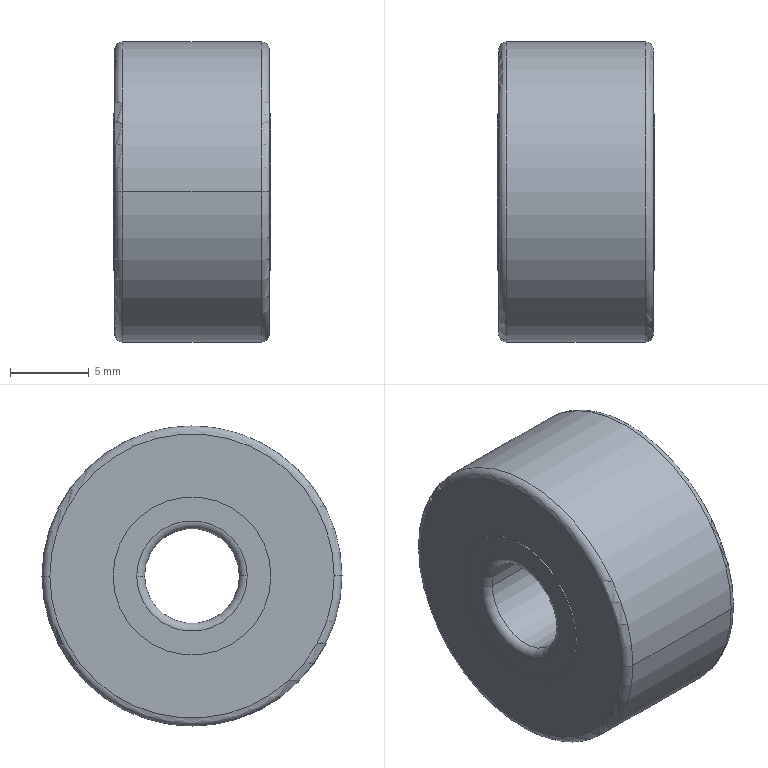Component | SolidWorks | ClampingArm2-1_BPS01-d6-1 | 1 solid | 20 faces | box 10 x 19 x 19 mm | volume 2503 mm3 | torus 8 | cylinder 8 | plane 4 | commonest cylinder face diameters 10 x4 6 x2 19 x2 | material Standard Part
build123d program:
from build123d import *

# Parameters (mm, degrees)
SKETCH1_R           = 9.5
BOSS_EXTRUDE1_DEPTH = 4.9
SKETCH2_R           = 5
BOSS_EXTRUDE2_DEPTH = 5
SKETCH3_R           = 3
CUT_EXTRUDE1_DEPTH  = 17.748
FILLET1_R           = 0.5


with BuildPart() as part:
    # Sketch1 → Boss-Extrude1 (new, symmetric)
    with BuildSketch(Plane(origin=(0, 0, 0), x_dir=(0, 0, -1), z_dir=(1, 0, 0))):
        Circle(SKETCH1_R)
    extrude(amount=BOSS_EXTRUDE1_DEPTH, both=True)

    # Sketch2 → Boss-Extrude2 (add, symmetric)
    with BuildSketch(Plane(origin=(0, 0, 0), x_dir=(0, 0, -1), z_dir=(1, 0, 0))):
        Circle(SKETCH2_R)
    extrude(amount=BOSS_EXTRUDE2_DEPTH, both=True)

    # Sketch3 → Cut-Extrude1 (cut, through all)
    with BuildSketch(Plane(origin=(5, 0, 0), x_dir=(0, 0, -1), z_dir=(1, 0, 0))):
        Circle(SKETCH3_R)
    extrude(amount=-CUT_EXTRUDE1_DEPTH, mode=Mode.SUBTRACT)

    # Fillet1
    fillet1_edges = [part.edges().sort_by_distance(p)[0] for p in [
        (-5, 0, 3),
        (5, 0, 3),
        (-4.9, 0, 9.5),
        (4.9, 0, 9.5),
    ]]
    fillet(fillet1_edges, radius=FILLET1_R)


solid = part.part

# Placed as in the assembly
solid = solid.moved(Location((-7.551, 66.046, -22.5), (0, 0, 0)))
STEP:
#1=COLOUR_RGB('',0.7922,0.8196,0.9333);
#2=FILL_AREA_STYLE_COLOUR('',#1);
#3=FILL_AREA_STYLE('',(#2));
#4=SURFACE_STYLE_FILL_AREA(#3);
#5=SURFACE_SIDE_STYLE('',(#4));
#6=SURFACE_STYLE_USAGE(.BOTH.,#5);
#7=PRESENTATION_STYLE_ASSIGNMENT((#6));
#8=CARTESIAN_POINT('',(-0.124,2.226,-0.8857));
#9=VERTEX_POINT('',#8);
#10=CARTESIAN_POINT('',(-0.124,2.974,-0.886));
#11=VERTEX_POINT('',#10);
#12=CARTESIAN_POINT('',(-0.124,2.6,-0.8858));
#13=DIRECTION('',(-1.,-0.,0.));
#14=DIRECTION('',(-0.,1.,-0.0003333));
#15=AXIS2_PLACEMENT_3D('',#12,#13,#14);
#16=CIRCLE('',#15,0.374);
#17=EDGE_CURVE('',#9,#11,#16,.T.);
#18=ORIENTED_EDGE('',*,*,#17,.F.);
#19=CARTESIAN_POINT('',(-0.1044,2.246,-0.8857));
#20=VERTEX_POINT('',#19);
#21=CARTESIAN_POINT('',(-0.124,2.246,-0.8857));
#22=DIRECTION('',(0.,0.0003333,1.));
#23=DIRECTION('',(0.,-1.,0.0003333));
#24=AXIS2_PLACEMENT_3D('',#21,#22,#23);
#25=CIRCLE('',#24,0.01969);
#26=EDGE_CURVE('',#9,#20,#25,.T.);
#27=ORIENTED_EDGE('',*,*,#26,.T.);
#28=CARTESIAN_POINT('',(-0.1044,2.955,-0.8859));
#29=VERTEX_POINT('',#28);
#30=CARTESIAN_POINT('',(-0.1044,2.6,-0.8858));
#31=DIRECTION('',(1.,0.,-0.));
#32=DIRECTION('',(-0.,1.,-0.0003333));
#33=AXIS2_PLACEMENT_3D('',#30,#31,#32);
#34=CIRCLE('',#33,0.3543);
#35=EDGE_CURVE('',#29,#20,#34,.T.);
#36=ORIENTED_EDGE('',*,*,#35,.F.);
#37=CARTESIAN_POINT('',(-0.124,2.955,-0.8859));
#38=DIRECTION('',(-0.,-0.0003333,-1.));
#39=DIRECTION('',(0.,1.,-0.0003333));
#40=AXIS2_PLACEMENT_3D('',#37,#38,#39);
#41=CIRCLE('',#40,0.01969);
#42=EDGE_CURVE('',#11,#29,#41,.T.);
#43=ORIENTED_EDGE('',*,*,#42,.F.);
#44=EDGE_LOOP('',(#18,#27,#36,#43));
#45=FACE_OUTER_BOUND('',#44,.T.);
#46=CARTESIAN_POINT('',(-0.124,2.6,-0.8858));
#47=DIRECTION('',(1.,0.,-0.));
#48=DIRECTION('',(-0.,1.,-0.0003333));
#49=AXIS2_PLACEMENT_3D('',#46,#47,#48);
#50=TOROIDAL_SURFACE('',#49,0.3543,0.01969);
#51=ADVANCED_FACE('',(#45),#50,.T.);
#52=CARTESIAN_POINT('',(-0.1004,2.462,-0.8858));
#53=VERTEX_POINT('',#52);
#54=CARTESIAN_POINT('',(-0.1004,2.738,-0.8859));
#55=VERTEX_POINT('',#54);
#56=CARTESIAN_POINT('',(-0.1004,2.6,-0.8858));
#57=DIRECTION('',(-1.,-0.,0.));
#58=DIRECTION('',(-0.,1.,-0.0003333));
#59=AXIS2_PLACEMENT_3D('',#56,#57,#58);
#60=CIRCLE('',#59,0.1378);
#61=EDGE_CURVE('',#53,#55,#60,.T.);
#62=ORIENTED_EDGE('',*,*,#61,.F.);
#63=CARTESIAN_POINT('',(-0.1201,2.482,-0.8858));
#64=VERTEX_POINT('',#63);
#65=CARTESIAN_POINT('',(-0.1201,2.462,-0.8858));
#66=DIRECTION('',(0.,0.0003333,1.));
#67=DIRECTION('',(0.,-1.,0.0003333));
#68=AXIS2_PLACEMENT_3D('',#65,#66,#67);
#69=CIRCLE('',#68,0.01969);
#70=EDGE_CURVE('',#53,#64,#69,.T.);
#71=ORIENTED_EDGE('',*,*,#70,.T.);
#72=CARTESIAN_POINT('',(-0.1201,2.718,-0.8859));
#73=VERTEX_POINT('',#72);
#74=CARTESIAN_POINT('',(-0.1201,2.6,-0.8858));
#75=DIRECTION('',(1.,0.,-0.));
#76=DIRECTION('',(-0.,1.,-0.0003333));
#77=AXIS2_PLACEMENT_3D('',#74,#75,#76);
#78=CIRCLE('',#77,0.1181);
#79=EDGE_CURVE('',#73,#64,#78,.T.);
#80=ORIENTED_EDGE('',*,*,#79,.F.);
#81=CARTESIAN_POINT('',(-0.1201,2.738,-0.8859));
#82=DIRECTION('',(-0.,-0.0003333,-1.));
#83=DIRECTION('',(0.,1.,-0.0003333));
#84=AXIS2_PLACEMENT_3D('',#81,#82,#83);
#85=CIRCLE('',#84,0.01969);
#86=EDGE_CURVE('',#55,#73,#85,.T.);
#87=ORIENTED_EDGE('',*,*,#86,.F.);
#88=EDGE_LOOP('',(#62,#71,#80,#87));
#89=FACE_OUTER_BOUND('',#88,.T.);
#90=CARTESIAN_POINT('',(-0.1201,2.6,-0.8858));
#91=DIRECTION('',(1.,0.,-0.));
#92=DIRECTION('',(-0.,1.,-0.0003333));
#93=AXIS2_PLACEMENT_3D('',#90,#91,#92);
#94=TOROIDAL_SURFACE('',#93,0.1378,0.01969);
#95=ADVANCED_FACE('',(#89),#94,.T.);
#96=CARTESIAN_POINT('',(-0.4902,2.246,-0.8857));
#97=VERTEX_POINT('',#96);
#98=CARTESIAN_POINT('',(-0.4902,2.955,-0.8859));
#99=VERTEX_POINT('',#98);
#100=CARTESIAN_POINT('',(-0.4902,2.6,-0.8858));
#101=DIRECTION('',(-1.,-0.,0.));
#102=DIRECTION('',(-0.,1.,-0.0003333));
#103=AXIS2_PLACEMENT_3D('',#100,#101,#102);
#104=CIRCLE('',#103,0.3543);
#105=EDGE_CURVE('',#97,#99,#104,.T.);
#106=ORIENTED_EDGE('',*,*,#105,.F.);
#107=CARTESIAN_POINT('',(-0.4705,2.226,-0.8857));
#108=VERTEX_POINT('',#107);
#109=CARTESIAN_POINT('',(-0.4705,2.246,-0.8857));
#110=DIRECTION('',(0.,0.0003333,1.));
#111=DIRECTION('',(0.,-1.,0.0003333));
#112=AXIS2_PLACEMENT_3D('',#109,#110,#111);
#113=CIRCLE('',#112,0.01969);
#114=EDGE_CURVE('',#97,#108,#113,.T.);
#115=ORIENTED_EDGE('',*,*,#114,.T.);
#116=CARTESIAN_POINT('',(-0.4705,2.974,-0.886));
#117=VERTEX_POINT('',#116);
#118=CARTESIAN_POINT('',(-0.4705,2.6,-0.8858));
#119=DIRECTION('',(1.,0.,-0.));
#120=DIRECTION('',(-0.,1.,-0.0003333));
#121=AXIS2_PLACEMENT_3D('',#118,#119,#120);
#122=CIRCLE('',#121,0.374);
#123=EDGE_CURVE('',#117,#108,#122,.T.);
#124=ORIENTED_EDGE('',*,*,#123,.F.);
#125=CARTESIAN_POINT('',(-0.4705,2.955,-0.8859));
#126=DIRECTION('',(-0.,-0.0003333,-1.));
#127=DIRECTION('',(0.,1.,-0.0003333));
#128=AXIS2_PLACEMENT_3D('',#125,#126,#127);
#129=CIRCLE('',#128,0.01969);
#130=EDGE_CURVE('',#99,#117,#129,.T.);
#131=ORIENTED_EDGE('',*,*,#130,.F.);
#132=EDGE_LOOP('',(#106,#115,#124,#131));
#133=FACE_OUTER_BOUND('',#132,.T.);
#134=CARTESIAN_POINT('',(-0.4705,2.6,-0.8858));
#135=DIRECTION('',(1.,0.,-0.));
#136=DIRECTION('',(-0.,1.,-0.0003333));
#137=AXIS2_PLACEMENT_3D('',#134,#135,#136);
#138=TOROIDAL_SURFACE('',#137,0.3543,0.01969);
#139=ADVANCED_FACE('',(#133),#138,.T.);
#140=CARTESIAN_POINT('',(-0.4744,2.482,-0.8858));
#141=VERTEX_POINT('',#140);
#142=CARTESIAN_POINT('',(-0.4744,2.718,-0.8859));
#143=VERTEX_POINT('',#142);
#144=CARTESIAN_POINT('',(-0.4744,2.6,-0.8858));
#145=DIRECTION('',(-1.,-0.,0.));
#146=DIRECTION('',(0.,1.,-0.0003333));
#147=AXIS2_PLACEMENT_3D('',#144,#145,#146);
#148=CIRCLE('',#147,0.1181);
#149=EDGE_CURVE('',#141,#143,#148,.T.);
#150=ORIENTED_EDGE('',*,*,#149,.F.);
#151=CARTESIAN_POINT('',(-0.4941,2.462,-0.8858));
#152=VERTEX_POINT('',#151);
#153=CARTESIAN_POINT('',(-0.4744,2.462,-0.8858));
#154=DIRECTION('',(0.,0.0003333,1.));
#155=DIRECTION('',(0.,-1.,0.0003333));
#156=AXIS2_PLACEMENT_3D('',#153,#154,#155);
#157=CIRCLE('',#156,0.01969);
#158=EDGE_CURVE('',#141,#152,#157,.T.);
#159=ORIENTED_EDGE('',*,*,#158,.T.);
#160=CARTESIAN_POINT('',(-0.4941,2.738,-0.8859));
#161=VERTEX_POINT('',#160);
#162=CARTESIAN_POINT('',(-0.4941,2.6,-0.8858));
#163=DIRECTION('',(1.,0.,-0.));
#164=DIRECTION('',(0.,1.,-0.0003333));
#165=AXIS2_PLACEMENT_3D('',#162,#163,#164);
#166=CIRCLE('',#165,0.1378);
#167=EDGE_CURVE('',#161,#152,#166,.T.);
#168=ORIENTED_EDGE('',*,*,#167,.F.);
#169=CARTESIAN_POINT('',(-0.4744,2.738,-0.8859));
#170=DIRECTION('',(-0.,-0.0003333,-1.));
#171=DIRECTION('',(0.,1.,-0.0003333));
#172=AXIS2_PLACEMENT_3D('',#169,#170,#171);
#173=CIRCLE('',#172,0.01969);
#174=EDGE_CURVE('',#143,#161,#173,.T.);
#175=ORIENTED_EDGE('',*,*,#174,.F.);
#176=EDGE_LOOP('',(#150,#159,#168,#175));
#177=FACE_OUTER_BOUND('',#176,.T.);
#178=CARTESIAN_POINT('',(-0.4744,2.6,-0.8858));
#179=DIRECTION('',(1.,0.,-0.));
#180=DIRECTION('',(-0.,1.,-0.0003333));
#181=AXIS2_PLACEMENT_3D('',#178,#179,#180);
#182=TOROIDAL_SURFACE('',#181,0.1378,0.01969);
#183=ADVANCED_FACE('',(#177),#182,.T.);
#184=CARTESIAN_POINT('',(-0.4744,2.6,-0.8858));
#185=DIRECTION('',(-1.,-0.,0.));
#186=DIRECTION('',(0.,1.,-0.0003333));
#187=AXIS2_PLACEMENT_3D('',#184,#185,#186);
#188=CIRCLE('',#187,0.1181);
#189=EDGE_CURVE('',#143,#141,#188,.T.);
#190=ORIENTED_EDGE('',*,*,#189,.T.);
#191=CARTESIAN_POINT('',(-0.4941,2.482,-0.8858));
#192=DIRECTION('',(1.,0.,-0.));
#193=VECTOR('',#192,39.37);
#194=LINE('',#191,#193);
#195=EDGE_CURVE('',#141,#64,#194,.T.);
#196=ORIENTED_EDGE('',*,*,#195,.T.);
#197=CARTESIAN_POINT('',(-0.1201,2.6,-0.8858));
#198=DIRECTION('',(1.,0.,-0.));
#199=DIRECTION('',(-0.,1.,-0.0003333));
#200=AXIS2_PLACEMENT_3D('',#197,#198,#199);
#201=CIRCLE('',#200,0.1181);
#202=EDGE_CURVE('',#64,#73,#201,.T.);
#203=ORIENTED_EDGE('',*,*,#202,.T.);
#204=CARTESIAN_POINT('',(-0.4941,2.718,-0.8859));
#205=DIRECTION('',(1.,0.,-0.));
#206=VECTOR('',#205,39.37);
#207=LINE('',#204,#206);
#208=EDGE_CURVE('',#143,#73,#207,.T.);
#209=ORIENTED_EDGE('',*,*,#208,.F.);
#210=EDGE_LOOP('',(#190,#196,#203,#209));
#211=FACE_OUTER_BOUND('',#210,.T.);
#212=CARTESIAN_POINT('',(-0.4941,2.6,-0.8858));
#213=DIRECTION('',(1.,0.,-0.));
#214=DIRECTION('',(0.,1.,-0.0003333));
#215=AXIS2_PLACEMENT_3D('',#212,#213,#214);
#216=CYLINDRICAL_SURFACE('',#215,0.1181);
#217=ADVANCED_FACE('',(#211),#216,.F.);
#218=CARTESIAN_POINT('',(-0.1004,2.797,-0.8859));
#219=VERTEX_POINT('',#218);
#220=CARTESIAN_POINT('',(-0.1004,2.403,-0.8858));
#221=VERTEX_POINT('',#220);
#222=CARTESIAN_POINT('',(-0.1004,2.6,-0.8858));
#223=DIRECTION('',(1.,0.,-0.));
#224=DIRECTION('',(-0.,1.,-0.0003333));
#225=AXIS2_PLACEMENT_3D('',#222,#223,#224);
#226=CIRCLE('',#225,0.1969);
#227=EDGE_CURVE('',#219,#221,#226,.T.);
#228=ORIENTED_EDGE('',*,*,#227,.F.);
#229=CARTESIAN_POINT('',(-0.1044,2.797,-0.8859));
#230=VERTEX_POINT('',#229);
#231=CARTESIAN_POINT('',(-0.1004,2.797,-0.8859));
#232=DIRECTION('',(-1.,-0.,0.));
#233=VECTOR('',#232,39.37);
#234=LINE('',#231,#233);
#235=EDGE_CURVE('',#219,#230,#234,.T.);
#236=ORIENTED_EDGE('',*,*,#235,.T.);
#237=CARTESIAN_POINT('',(-0.1044,2.403,-0.8858));
#238=VERTEX_POINT('',#237);
#239=CARTESIAN_POINT('',(-0.1044,2.6,-0.8858));
#240=DIRECTION('',(-1.,-0.,0.));
#241=DIRECTION('',(-0.,1.,-0.0003333));
#242=AXIS2_PLACEMENT_3D('',#239,#240,#241);
#243=CIRCLE('',#242,0.1969);
#244=EDGE_CURVE('',#238,#230,#243,.T.);
#245=ORIENTED_EDGE('',*,*,#244,.F.);
#246=CARTESIAN_POINT('',(-0.1004,2.403,-0.8858));
#247=DIRECTION('',(-1.,-0.,0.));
#248=VECTOR('',#247,39.37);
#249=LINE('',#246,#248);
#250=EDGE_CURVE('',#221,#238,#249,.T.);
#251=ORIENTED_EDGE('',*,*,#250,.F.);
#252=EDGE_LOOP('',(#228,#236,#245,#251));
#253=FACE_OUTER_BOUND('',#252,.T.);
#254=CARTESIAN_POINT('',(-0.1004,2.6,-0.8858));
#255=DIRECTION('',(-1.,-0.,0.));
#256=DIRECTION('',(0.,-1.,0.0003333));
#257=AXIS2_PLACEMENT_3D('',#254,#255,#256);
#258=CYLINDRICAL_SURFACE('',#257,0.1969);
#259=ADVANCED_FACE('',(#253),#258,.T.);
#260=CARTESIAN_POINT('',(-0.4902,2.403,-0.8858));
#261=VERTEX_POINT('',#260);
#262=CARTESIAN_POINT('',(-0.4902,2.797,-0.8859));
#263=VERTEX_POINT('',#262);
#264=CARTESIAN_POINT('',(-0.4902,2.6,-0.8858));
#265=DIRECTION('',(-1.,-0.,0.));
#266=DIRECTION('',(-0.,1.,-0.0003333));
#267=AXIS2_PLACEMENT_3D('',#264,#265,#266);
#268=CIRCLE('',#267,0.1969);
#269=EDGE_CURVE('',#261,#263,#268,.T.);
#270=ORIENTED_EDGE('',*,*,#269,.T.);
#271=CARTESIAN_POINT('',(-0.4941,2.797,-0.8859));
#272=VERTEX_POINT('',#271);
#273=CARTESIAN_POINT('',(-0.1004,2.797,-0.8859));
#274=DIRECTION('',(-1.,-0.,0.));
#275=VECTOR('',#274,39.37);
#276=LINE('',#273,#275);
#277=EDGE_CURVE('',#263,#272,#276,.T.);
#278=ORIENTED_EDGE('',*,*,#277,.T.);
#279=CARTESIAN_POINT('',(-0.4941,2.403,-0.8858));
#280=VERTEX_POINT('',#279);
#281=CARTESIAN_POINT('',(-0.4941,2.6,-0.8858));
#282=DIRECTION('',(1.,0.,-0.));
#283=DIRECTION('',(-0.,1.,-0.0003333));
#284=AXIS2_PLACEMENT_3D('',#281,#282,#283);
#285=CIRCLE('',#284,0.1969);
#286=EDGE_CURVE('',#272,#280,#285,.T.);
#287=ORIENTED_EDGE('',*,*,#286,.T.);
#288=CARTESIAN_POINT('',(-0.1004,2.403,-0.8858));
#289=DIRECTION('',(-1.,-0.,0.));
#290=VECTOR('',#289,39.37);
#291=LINE('',#288,#290);
#292=EDGE_CURVE('',#261,#280,#291,.T.);
#293=ORIENTED_EDGE('',*,*,#292,.F.);
#294=EDGE_LOOP('',(#270,#278,#287,#293));
#295=FACE_OUTER_BOUND('',#294,.T.);
#296=CARTESIAN_POINT('',(-0.1004,2.6,-0.8858));
#297=DIRECTION('',(-1.,-0.,0.));
#298=DIRECTION('',(0.,-1.,0.0003333));
#299=AXIS2_PLACEMENT_3D('',#296,#297,#298);
#300=CYLINDRICAL_SURFACE('',#299,0.1969);
#301=ADVANCED_FACE('',(#295),#300,.T.);
#302=ORIENTED_EDGE('',*,*,#17,.T.);
#303=CARTESIAN_POINT('',(-0.1044,2.974,-0.886));
#304=DIRECTION('',(-1.,-0.,0.));
#305=VECTOR('',#304,39.37);
#306=LINE('',#303,#305);
#307=EDGE_CURVE('',#11,#117,#306,.T.);
#308=ORIENTED_EDGE('',*,*,#307,.T.);
#309=ORIENTED_EDGE('',*,*,#123,.T.);
#310=CARTESIAN_POINT('',(-0.1044,2.226,-0.8857));
#311=DIRECTION('',(-1.,-0.,0.));
#312=VECTOR('',#311,39.37);
#313=LINE('',#310,#312);
#314=EDGE_CURVE('',#9,#108,#313,.T.);
#315=ORIENTED_EDGE('',*,*,#314,.F.);
#316=EDGE_LOOP('',(#302,#308,#309,#315));
#317=FACE_OUTER_BOUND('',#316,.T.);
#318=CARTESIAN_POINT('',(-0.1044,2.6,-0.8858));
#319=DIRECTION('',(-1.,-0.,0.));
#320=DIRECTION('',(0.,-1.,0.0003333));
#321=AXIS2_PLACEMENT_3D('',#318,#319,#320);
#322=CYLINDRICAL_SURFACE('',#321,0.374);
#323=ADVANCED_FACE('',(#317),#322,.T.);
#324=ORIENTED_EDGE('',*,*,#307,.F.);
#325=CARTESIAN_POINT('',(-0.124,2.6,-0.8858));
#326=DIRECTION('',(-1.,-0.,0.));
#327=DIRECTION('',(-0.,1.,-0.0003333));
#328=AXIS2_PLACEMENT_3D('',#325,#326,#327);
#329=CIRCLE('',#328,0.374);
#330=EDGE_CURVE('',#11,#9,#329,.T.);
#331=ORIENTED_EDGE('',*,*,#330,.T.);
#332=ORIENTED_EDGE('',*,*,#314,.T.);
#333=CARTESIAN_POINT('',(-0.4705,2.6,-0.8858));
#334=DIRECTION('',(1.,0.,-0.));
#335=DIRECTION('',(-0.,1.,-0.0003333));
#336=AXIS2_PLACEMENT_3D('',#333,#334,#335);
#337=CIRCLE('',#336,0.374);
#338=EDGE_CURVE('',#108,#117,#337,.T.);
#339=ORIENTED_EDGE('',*,*,#338,.T.);
#340=EDGE_LOOP('',(#324,#331,#332,#339));
#341=FACE_OUTER_BOUND('',#340,.T.);
#342=CARTESIAN_POINT('',(-0.1044,2.6,-0.8858));
#343=DIRECTION('',(-1.,-0.,0.));
#344=DIRECTION('',(0.,-1.,0.0003333));
#345=AXIS2_PLACEMENT_3D('',#342,#343,#344);
#346=CYLINDRICAL_SURFACE('',#345,0.374);
#347=ADVANCED_FACE('',(#341),#346,.T.);
#348=ORIENTED_EDGE('',*,*,#35,.T.);
#349=CARTESIAN_POINT('',(-0.1044,2.6,-0.8858));
#350=DIRECTION('',(1.,0.,-0.));
#351=DIRECTION('',(-0.,1.,-0.0003333));
#352=AXIS2_PLACEMENT_3D('',#349,#350,#351);
#353=CIRCLE('',#352,0.3543);
#354=EDGE_CURVE('',#20,#29,#353,.T.);
#355=ORIENTED_EDGE('',*,*,#354,.T.);
#356=EDGE_LOOP('',(#348,#355));
#357=FACE_OUTER_BOUND('',#356,.T.);
#358=ORIENTED_EDGE('',*,*,#244,.T.);
#359=CARTESIAN_POINT('',(-0.1044,2.6,-0.8858));
#360=DIRECTION('',(-1.,-0.,0.));
#361=DIRECTION('',(-0.,1.,-0.0003333));
#362=AXIS2_PLACEMENT_3D('',#359,#360,#361);
#363=CIRCLE('',#362,0.1969);
#364=EDGE_CURVE('',#230,#238,#363,.T.);
#365=ORIENTED_EDGE('',*,*,#364,.T.);
#366=EDGE_LOOP('',(#358,#365));
#367=FACE_BOUND('',#366,.T.);
#368=CARTESIAN_POINT('',(-0.1044,2.6,-0.8858));
#369=DIRECTION('',(1.,0.,-0.));
#370=DIRECTION('',(-0.,1.,-0.0003333));
#371=AXIS2_PLACEMENT_3D('',#368,#369,#370);
#372=PLANE('',#371);
#373=ADVANCED_FACE('',(#357,#367),#372,.T.);
#374=CARTESIAN_POINT('',(-0.4902,2.6,-0.8858));
#375=DIRECTION('',(-1.,-0.,0.));
#376=DIRECTION('',(-0.,1.,-0.0003333));
#377=AXIS2_PLACEMENT_3D('',#374,#375,#376);
#378=CIRCLE('',#377,0.3543);
#379=EDGE_CURVE('',#99,#97,#378,.T.);
#380=ORIENTED_EDGE('',*,*,#379,.T.);
#381=ORIENTED_EDGE('',*,*,#105,.T.);
#382=EDGE_LOOP('',(#380,#381));
#383=FACE_OUTER_BOUND('',#382,.T.);
#384=ORIENTED_EDGE('',*,*,#269,.F.);
#385=CARTESIAN_POINT('',(-0.4902,2.6,-0.8858));
#386=DIRECTION('',(-1.,-0.,0.));
#387=DIRECTION('',(-0.,1.,-0.0003333));
#388=AXIS2_PLACEMENT_3D('',#385,#386,#387);
#389=CIRCLE('',#388,0.1969);
#390=EDGE_CURVE('',#263,#261,#389,.T.);
#391=ORIENTED_EDGE('',*,*,#390,.F.);
#392=EDGE_LOOP('',(#384,#391));
#393=FACE_BOUND('',#392,.T.);
#394=CARTESIAN_POINT('',(-0.4902,2.6,-0.8858));
#395=DIRECTION('',(1.,0.,-0.));
#396=DIRECTION('',(-0.,1.,-0.0003333));
#397=AXIS2_PLACEMENT_3D('',#394,#395,#396);
#398=PLANE('',#397);
#399=ADVANCED_FACE('',(#383,#393),#398,.F.);
#400=ORIENTED_EDGE('',*,*,#167,.T.);
#401=CARTESIAN_POINT('',(-0.4941,2.6,-0.8858));
#402=DIRECTION('',(1.,0.,-0.));
#403=DIRECTION('',(0.,1.,-0.0003333));
#404=AXIS2_PLACEMENT_3D('',#401,#402,#403);
#405=CIRCLE('',#404,0.1378);
#406=EDGE_CURVE('',#152,#161,#405,.T.);
#407=ORIENTED_EDGE('',*,*,#406,.T.);
#408=EDGE_LOOP('',(#400,#407));
#409=FACE_BOUND('',#408,.T.);
#410=CARTESIAN_POINT('',(-0.4941,2.6,-0.8858));
#411=DIRECTION('',(1.,0.,-0.));
#412=DIRECTION('',(-0.,1.,-0.0003333));
#413=AXIS2_PLACEMENT_3D('',#410,#411,#412);
#414=CIRCLE('',#413,0.1969);
#415=EDGE_CURVE('',#280,#272,#414,.T.);
#416=ORIENTED_EDGE('',*,*,#415,.F.);
#417=ORIENTED_EDGE('',*,*,#286,.F.);
#418=EDGE_LOOP('',(#416,#417));
#419=FACE_OUTER_BOUND('',#418,.T.);
#420=CARTESIAN_POINT('',(-0.4941,2.6,-0.8858));
#421=DIRECTION('',(1.,0.,-0.));
#422=DIRECTION('',(-0.,1.,-0.0003333));
#423=AXIS2_PLACEMENT_3D('',#420,#421,#422);
#424=PLANE('',#423);
#425=ADVANCED_FACE('',(#409,#419),#424,.F.);
#426=ORIENTED_EDGE('',*,*,#277,.F.);
#427=ORIENTED_EDGE('',*,*,#390,.T.);
#428=ORIENTED_EDGE('',*,*,#292,.T.);
#429=ORIENTED_EDGE('',*,*,#415,.T.);
#430=EDGE_LOOP('',(#426,#427,#428,#429));
#431=FACE_OUTER_BOUND('',#430,.T.);
#432=CARTESIAN_POINT('',(-0.1004,2.6,-0.8858));
#433=DIRECTION('',(-1.,-0.,0.));
#434=DIRECTION('',(0.,-1.,0.0003333));
#435=AXIS2_PLACEMENT_3D('',#432,#433,#434);
#436=CYLINDRICAL_SURFACE('',#435,0.1969);
#437=ADVANCED_FACE('',(#431),#436,.T.);
#438=ORIENTED_EDGE('',*,*,#235,.F.);
#439=CARTESIAN_POINT('',(-0.1004,2.6,-0.8858));
#440=DIRECTION('',(1.,0.,-0.));
#441=DIRECTION('',(-0.,1.,-0.0003333));
#442=AXIS2_PLACEMENT_3D('',#439,#440,#441);
#443=CIRCLE('',#442,0.1969);
#444=EDGE_CURVE('',#221,#219,#443,.T.);
#445=ORIENTED_EDGE('',*,*,#444,.F.);
#446=ORIENTED_EDGE('',*,*,#250,.T.);
#447=ORIENTED_EDGE('',*,*,#364,.F.);
#448=EDGE_LOOP('',(#438,#445,#446,#447));
#449=FACE_OUTER_BOUND('',#448,.T.);
#450=CARTESIAN_POINT('',(-0.1004,2.6,-0.8858));
#451=DIRECTION('',(-1.,-0.,0.));
#452=DIRECTION('',(0.,-1.,0.0003333));
#453=AXIS2_PLACEMENT_3D('',#450,#451,#452);
#454=CYLINDRICAL_SURFACE('',#453,0.1969);
#455=ADVANCED_FACE('',(#449),#454,.T.);
#456=CARTESIAN_POINT('',(-0.1004,2.6,-0.8858));
#457=DIRECTION('',(-1.,-0.,0.));
#458=DIRECTION('',(-0.,1.,-0.0003333));
#459=AXIS2_PLACEMENT_3D('',#456,#457,#458);
#460=CIRCLE('',#459,0.1378);
#461=EDGE_CURVE('',#55,#53,#460,.T.);
#462=ORIENTED_EDGE('',*,*,#461,.T.);
#463=ORIENTED_EDGE('',*,*,#61,.T.);
#464=EDGE_LOOP('',(#462,#463));
#465=FACE_BOUND('',#464,.T.);
#466=ORIENTED_EDGE('',*,*,#444,.T.);
#467=ORIENTED_EDGE('',*,*,#227,.T.);
#468=EDGE_LOOP('',(#466,#467));
#469=FACE_OUTER_BOUND('',#468,.T.);
#470=CARTESIAN_POINT('',(-0.1004,2.6,-0.8858));
#471=DIRECTION('',(1.,0.,-0.));
#472=DIRECTION('',(-0.,1.,-0.0003333));
#473=AXIS2_PLACEMENT_3D('',#470,#471,#472);
#474=PLANE('',#473);
#475=ADVANCED_FACE('',(#465,#469),#474,.T.);
#476=ORIENTED_EDGE('',*,*,#195,.F.);
#477=ORIENTED_EDGE('',*,*,#149,.T.);
#478=ORIENTED_EDGE('',*,*,#208,.T.);
#479=ORIENTED_EDGE('',*,*,#79,.T.);
#480=EDGE_LOOP('',(#476,#477,#478,#479));
#481=FACE_OUTER_BOUND('',#480,.T.);
#482=CARTESIAN_POINT('',(-0.4941,2.6,-0.8858));
#483=DIRECTION('',(1.,0.,-0.));
#484=DIRECTION('',(0.,1.,-0.0003333));
#485=AXIS2_PLACEMENT_3D('',#482,#483,#484);
#486=CYLINDRICAL_SURFACE('',#485,0.1181);
#487=ADVANCED_FACE('',(#481),#486,.F.);
#488=ORIENTED_EDGE('',*,*,#158,.F.);
#489=ORIENTED_EDGE('',*,*,#189,.F.);
#490=ORIENTED_EDGE('',*,*,#174,.T.);
#491=ORIENTED_EDGE('',*,*,#406,.F.);
#492=EDGE_LOOP('',(#488,#489,#490,#491));
#493=FACE_OUTER_BOUND('',#492,.T.);
#494=CARTESIAN_POINT('',(-0.4744,2.6,-0.8858));
#495=DIRECTION('',(1.,0.,-0.));
#496=DIRECTION('',(-0.,1.,-0.0003333));
#497=AXIS2_PLACEMENT_3D('',#494,#495,#496);
#498=TOROIDAL_SURFACE('',#497,0.1378,0.01969);
#499=ADVANCED_FACE('',(#493),#498,.T.);
#500=ORIENTED_EDGE('',*,*,#114,.F.);
#501=ORIENTED_EDGE('',*,*,#379,.F.);
#502=ORIENTED_EDGE('',*,*,#130,.T.);
#503=ORIENTED_EDGE('',*,*,#338,.F.);
#504=EDGE_LOOP('',(#500,#501,#502,#503));
#505=FACE_OUTER_BOUND('',#504,.T.);
#506=CARTESIAN_POINT('',(-0.4705,2.6,-0.8858));
#507=DIRECTION('',(1.,0.,-0.));
#508=DIRECTION('',(-0.,1.,-0.0003333));
#509=AXIS2_PLACEMENT_3D('',#506,#507,#508);
#510=TOROIDAL_SURFACE('',#509,0.3543,0.01969);
#511=ADVANCED_FACE('',(#505),#510,.T.);
#512=ORIENTED_EDGE('',*,*,#70,.F.);
#513=ORIENTED_EDGE('',*,*,#461,.F.);
#514=ORIENTED_EDGE('',*,*,#86,.T.);
#515=ORIENTED_EDGE('',*,*,#202,.F.);
#516=EDGE_LOOP('',(#512,#513,#514,#515));
#517=FACE_OUTER_BOUND('',#516,.T.);
#518=CARTESIAN_POINT('',(-0.1201,2.6,-0.8858));
#519=DIRECTION('',(1.,0.,-0.));
#520=DIRECTION('',(-0.,1.,-0.0003333));
#521=AXIS2_PLACEMENT_3D('',#518,#519,#520);
#522=TOROIDAL_SURFACE('',#521,0.1378,0.01969);
#523=ADVANCED_FACE('',(#517),#522,.T.);
#524=ORIENTED_EDGE('',*,*,#26,.F.);
#525=ORIENTED_EDGE('',*,*,#330,.F.);
#526=ORIENTED_EDGE('',*,*,#42,.T.);
#527=ORIENTED_EDGE('',*,*,#354,.F.);
#528=EDGE_LOOP('',(#524,#525,#526,#527));
#529=FACE_OUTER_BOUND('',#528,.T.);
#530=CARTESIAN_POINT('',(-0.124,2.6,-0.8858));
#531=DIRECTION('',(1.,0.,-0.));
#532=DIRECTION('',(-0.,1.,-0.0003333));
#533=AXIS2_PLACEMENT_3D('',#530,#531,#532);
#534=TOROIDAL_SURFACE('',#533,0.3543,0.01969);
#535=ADVANCED_FACE('',(#529),#534,.T.);
#536=CLOSED_SHELL('',(#51,#95,#139,#183,#217,#259,#301,#323,#347,#373,#399,#425,#437,#455,#475,#487,#499,#511,#523,#535));
#537=MANIFOLD_SOLID_BREP('',#536);
#538=STYLED_ITEM('',(#7),#537);
#539=(LENGTH_UNIT()NAMED_UNIT(*)SI_UNIT($,.METRE.));
#540=LENGTH_MEASURE_WITH_UNIT(LENGTH_MEASURE(0.0254),#539);
#541=DIMENSIONAL_EXPONENTS(1.,0.,0.,0.,0.,0.,0.);
#542=(CONVERSION_BASED_UNIT('',#540)LENGTH_UNIT()NAMED_UNIT(#541));
#543=UNCERTAINTY_MEASURE_WITH_UNIT(LENGTH_MEASURE(0.00001),#542,'','');
#544=(NAMED_UNIT(*)PLANE_ANGLE_UNIT()SI_UNIT($,.RADIAN.));
#545=(NAMED_UNIT(*)SI_UNIT($,.STERADIAN.)SOLID_ANGLE_UNIT());
#546=(GEOMETRIC_REPRESENTATION_CONTEXT(3)GLOBAL_UNCERTAINTY_ASSIGNED_CONTEXT((#543))GLOBAL_UNIT_ASSIGNED_CONTEXT((#542,#544,#545))REPRESENTATION_CONTEXT('',''));
#547=MECHANICAL_DESIGN_GEOMETRIC_PRESENTATION_REPRESENTATION('',(#538),#546);
#548=CARTESIAN_POINT('',(0.,0.,0.));
#549=DIRECTION('',(0.,0.,1.));
#550=DIRECTION('',(1.,0.,0.));
#551=AXIS2_PLACEMENT_3D('',#548,#549,#550);
#552=(LENGTH_UNIT()NAMED_UNIT(*)SI_UNIT($,.METRE.));
#553=LENGTH_MEASURE_WITH_UNIT(LENGTH_MEASURE(0.0254),#552);
#554=DIMENSIONAL_EXPONENTS(1.,0.,0.,0.,0.,0.,0.);
#555=(CONVERSION_BASED_UNIT('',#553)LENGTH_UNIT()NAMED_UNIT(#554));
#556=UNCERTAINTY_MEASURE_WITH_UNIT(LENGTH_MEASURE(0.00001),#555,'','');
#557=(NAMED_UNIT(*)PLANE_ANGLE_UNIT()SI_UNIT($,.RADIAN.));
#558=(NAMED_UNIT(*)SI_UNIT($,.STERADIAN.)SOLID_ANGLE_UNIT());
#559=(GEOMETRIC_REPRESENTATION_CONTEXT(3)GLOBAL_UNCERTAINTY_ASSIGNED_CONTEXT((#556))GLOBAL_UNIT_ASSIGNED_CONTEXT((#555,#557,#558))REPRESENTATION_CONTEXT('',''));
#560=ADVANCED_BREP_SHAPE_REPRESENTATION('',(#537,#551),#559);
#561=PRESENTATION_LAYER_ASSIGNMENT('','',(#538));